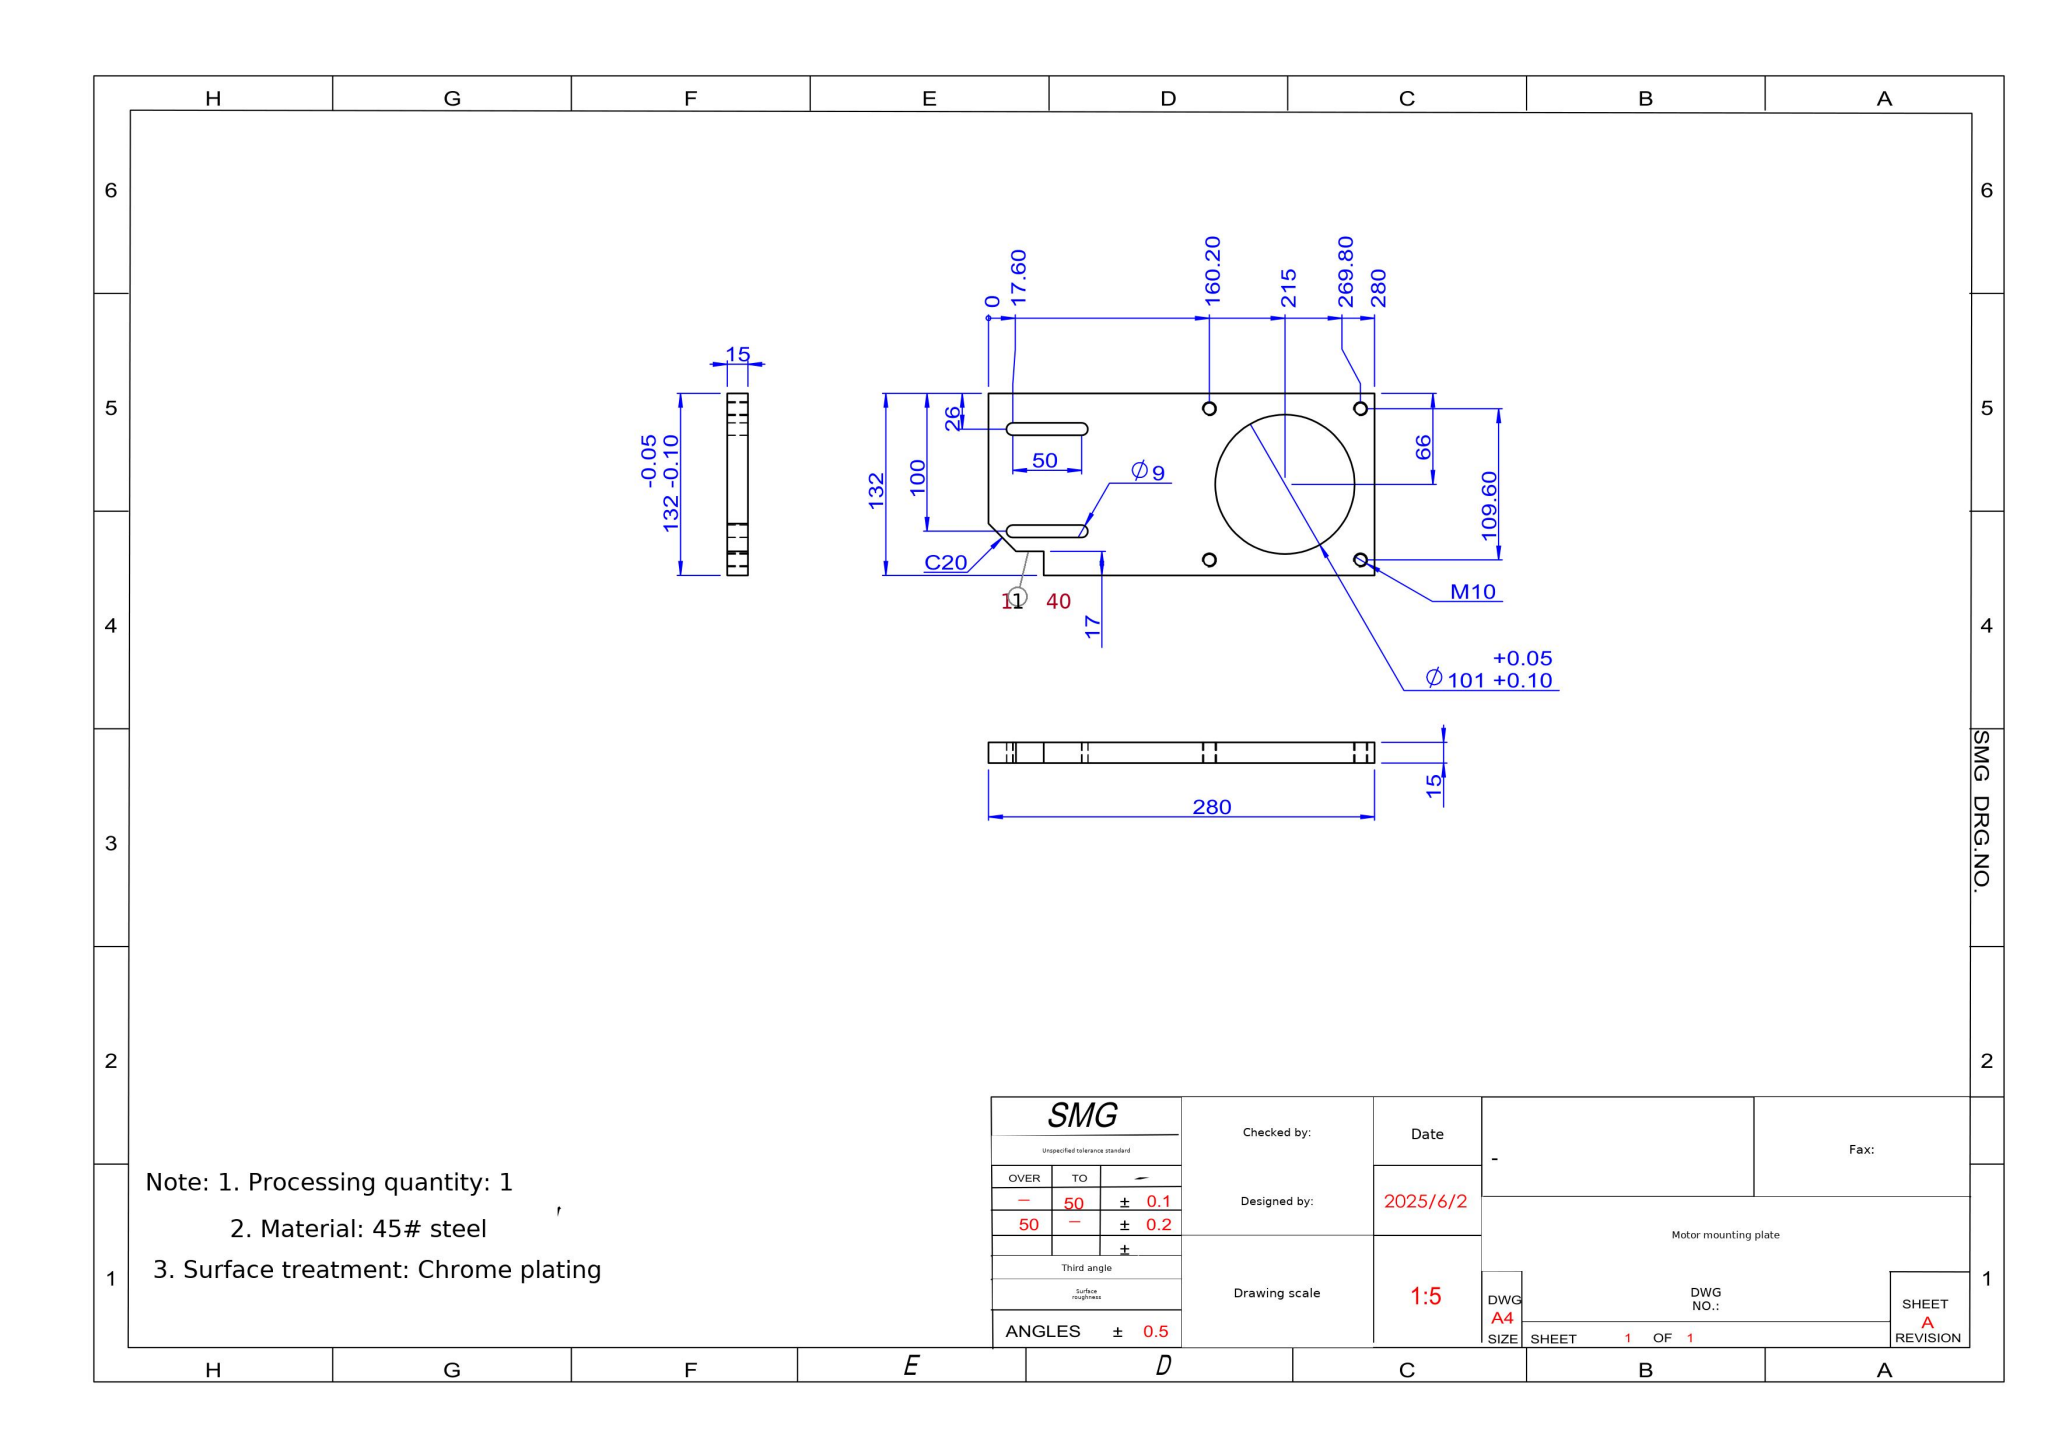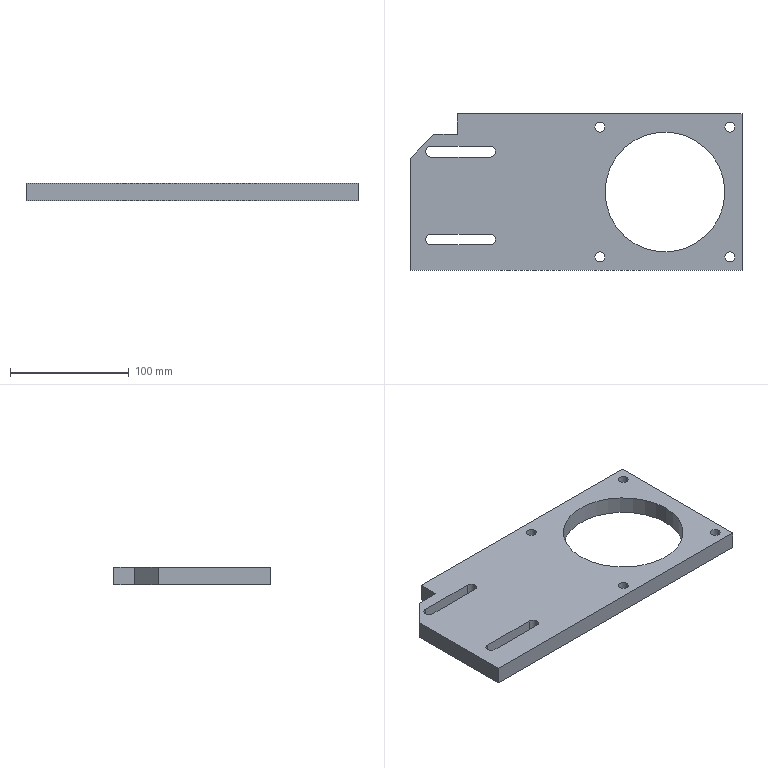Part | SolidWorks | mm | material 45# steel | 1 solid | 29 faces | box 280 x 132 x 15 mm | volume 401909 mm3 | cylinder 16 | plane 13 | commonest cylinder face diameters 8.5 x8 9 x6 101 x2
STEP:
#1=CARTESIAN_POINT('',(15.949,54.801,0.));
#2=VERTEX_POINT('',#1);
#3=CARTESIAN_POINT('',(24.449,54.801,0.));
#4=VERTEX_POINT('',#3);
#5=CARTESIAN_POINT('',(20.199,54.801,0.));
#6=DIRECTION('',(0.,0.,1.));
#7=DIRECTION('',(1.,0.,0.));
#8=AXIS2_PLACEMENT_3D('',#5,#6,#7);
#9=CIRCLE('',#8,4.25);
#10=EDGE_CURVE('',#2,#4,#9,.T.);
#11=ORIENTED_EDGE('',*,*,#10,.F.);
#12=CARTESIAN_POINT('',(15.949,54.801,15.));
#13=VERTEX_POINT('',#12);
#14=CARTESIAN_POINT('',(15.949,54.801,15.));
#15=DIRECTION('',(0.,0.,1.));
#16=VECTOR('',#15,1000.);
#17=LINE('',#14,#16);
#18=EDGE_CURVE('',#2,#13,#17,.T.);
#19=ORIENTED_EDGE('',*,*,#18,.T.);
#20=CARTESIAN_POINT('',(24.449,54.801,15.));
#21=VERTEX_POINT('',#20);
#22=CARTESIAN_POINT('',(20.199,54.801,15.));
#23=DIRECTION('',(0.,0.,-1.));
#24=DIRECTION('',(1.,0.,0.));
#25=AXIS2_PLACEMENT_3D('',#22,#23,#24);
#26=CIRCLE('',#25,4.25);
#27=EDGE_CURVE('',#21,#13,#26,.T.);
#28=ORIENTED_EDGE('',*,*,#27,.F.);
#29=CARTESIAN_POINT('',(24.449,54.801,15.));
#30=DIRECTION('',(0.,0.,1.));
#31=VECTOR('',#30,1000.);
#32=LINE('',#29,#31);
#33=EDGE_CURVE('',#4,#21,#32,.T.);
#34=ORIENTED_EDGE('',*,*,#33,.F.);
#35=EDGE_LOOP('',(#11,#19,#28,#34));
#36=FACE_OUTER_BOUND('',#35,.T.);
#37=CARTESIAN_POINT('',(20.199,54.801,15.));
#38=DIRECTION('',(0.,0.,1.));
#39=DIRECTION('',(1.,0.,0.));
#40=AXIS2_PLACEMENT_3D('',#37,#38,#39);
#41=CYLINDRICAL_SURFACE('',#40,4.25);
#42=ADVANCED_FACE('',(#36),#41,.F.);
#43=CARTESIAN_POINT('',(15.949,-54.801,0.));
#44=VERTEX_POINT('',#43);
#45=CARTESIAN_POINT('',(24.449,-54.801,0.));
#46=VERTEX_POINT('',#45);
#47=CARTESIAN_POINT('',(20.199,-54.801,0.));
#48=DIRECTION('',(0.,0.,1.));
#49=DIRECTION('',(1.,0.,0.));
#50=AXIS2_PLACEMENT_3D('',#47,#48,#49);
#51=CIRCLE('',#50,4.25);
#52=EDGE_CURVE('',#44,#46,#51,.T.);
#53=ORIENTED_EDGE('',*,*,#52,.F.);
#54=CARTESIAN_POINT('',(15.949,-54.801,15.));
#55=VERTEX_POINT('',#54);
#56=CARTESIAN_POINT('',(15.949,-54.801,15.));
#57=DIRECTION('',(0.,0.,1.));
#58=VECTOR('',#57,1000.);
#59=LINE('',#56,#58);
#60=EDGE_CURVE('',#44,#55,#59,.T.);
#61=ORIENTED_EDGE('',*,*,#60,.T.);
#62=CARTESIAN_POINT('',(24.449,-54.801,15.));
#63=VERTEX_POINT('',#62);
#64=CARTESIAN_POINT('',(20.199,-54.801,15.));
#65=DIRECTION('',(0.,0.,-1.));
#66=DIRECTION('',(1.,0.,0.));
#67=AXIS2_PLACEMENT_3D('',#64,#65,#66);
#68=CIRCLE('',#67,4.25);
#69=EDGE_CURVE('',#63,#55,#68,.T.);
#70=ORIENTED_EDGE('',*,*,#69,.F.);
#71=CARTESIAN_POINT('',(24.449,-54.801,15.));
#72=DIRECTION('',(0.,0.,1.));
#73=VECTOR('',#72,1000.);
#74=LINE('',#71,#73);
#75=EDGE_CURVE('',#46,#63,#74,.T.);
#76=ORIENTED_EDGE('',*,*,#75,.F.);
#77=EDGE_LOOP('',(#53,#61,#70,#76));
#78=FACE_OUTER_BOUND('',#77,.T.);
#79=CARTESIAN_POINT('',(20.199,-54.801,15.));
#80=DIRECTION('',(0.,0.,1.));
#81=DIRECTION('',(1.,0.,0.));
#82=AXIS2_PLACEMENT_3D('',#79,#80,#81);
#83=CYLINDRICAL_SURFACE('',#82,4.25);
#84=ADVANCED_FACE('',(#78),#83,.F.);
#85=CARTESIAN_POINT('',(125.551,-54.801,0.));
#86=VERTEX_POINT('',#85);
#87=CARTESIAN_POINT('',(134.051,-54.801,0.));
#88=VERTEX_POINT('',#87);
#89=CARTESIAN_POINT('',(129.801,-54.801,0.));
#90=DIRECTION('',(0.,0.,1.));
#91=DIRECTION('',(1.,0.,0.));
#92=AXIS2_PLACEMENT_3D('',#89,#90,#91);
#93=CIRCLE('',#92,4.25);
#94=EDGE_CURVE('',#86,#88,#93,.T.);
#95=ORIENTED_EDGE('',*,*,#94,.F.);
#96=CARTESIAN_POINT('',(125.551,-54.801,15.));
#97=VERTEX_POINT('',#96);
#98=CARTESIAN_POINT('',(125.551,-54.801,15.));
#99=DIRECTION('',(0.,0.,1.));
#100=VECTOR('',#99,1000.);
#101=LINE('',#98,#100);
#102=EDGE_CURVE('',#86,#97,#101,.T.);
#103=ORIENTED_EDGE('',*,*,#102,.T.);
#104=CARTESIAN_POINT('',(134.051,-54.801,15.));
#105=VERTEX_POINT('',#104);
#106=CARTESIAN_POINT('',(129.801,-54.801,15.));
#107=DIRECTION('',(0.,0.,-1.));
#108=DIRECTION('',(1.,0.,0.));
#109=AXIS2_PLACEMENT_3D('',#106,#107,#108);
#110=CIRCLE('',#109,4.25);
#111=EDGE_CURVE('',#105,#97,#110,.T.);
#112=ORIENTED_EDGE('',*,*,#111,.F.);
#113=CARTESIAN_POINT('',(134.051,-54.801,15.));
#114=DIRECTION('',(0.,0.,1.));
#115=VECTOR('',#114,1000.);
#116=LINE('',#113,#115);
#117=EDGE_CURVE('',#88,#105,#116,.T.);
#118=ORIENTED_EDGE('',*,*,#117,.F.);
#119=EDGE_LOOP('',(#95,#103,#112,#118));
#120=FACE_OUTER_BOUND('',#119,.T.);
#121=CARTESIAN_POINT('',(129.801,-54.801,15.));
#122=DIRECTION('',(0.,0.,1.));
#123=DIRECTION('',(1.,0.,0.));
#124=AXIS2_PLACEMENT_3D('',#121,#122,#123);
#125=CYLINDRICAL_SURFACE('',#124,4.25);
#126=ADVANCED_FACE('',(#120),#125,.F.);
#127=CARTESIAN_POINT('',(125.551,54.801,0.));
#128=VERTEX_POINT('',#127);
#129=CARTESIAN_POINT('',(134.051,54.801,0.));
#130=VERTEX_POINT('',#129);
#131=CARTESIAN_POINT('',(129.801,54.801,0.));
#132=DIRECTION('',(0.,0.,1.));
#133=DIRECTION('',(1.,0.,0.));
#134=AXIS2_PLACEMENT_3D('',#131,#132,#133);
#135=CIRCLE('',#134,4.25);
#136=EDGE_CURVE('',#128,#130,#135,.T.);
#137=ORIENTED_EDGE('',*,*,#136,.F.);
#138=CARTESIAN_POINT('',(125.551,54.801,15.));
#139=VERTEX_POINT('',#138);
#140=CARTESIAN_POINT('',(125.551,54.801,15.));
#141=DIRECTION('',(0.,0.,1.));
#142=VECTOR('',#141,1000.);
#143=LINE('',#140,#142);
#144=EDGE_CURVE('',#128,#139,#143,.T.);
#145=ORIENTED_EDGE('',*,*,#144,.T.);
#146=CARTESIAN_POINT('',(134.051,54.801,15.));
#147=VERTEX_POINT('',#146);
#148=CARTESIAN_POINT('',(129.801,54.801,15.));
#149=DIRECTION('',(0.,0.,-1.));
#150=DIRECTION('',(1.,0.,0.));
#151=AXIS2_PLACEMENT_3D('',#148,#149,#150);
#152=CIRCLE('',#151,4.25);
#153=EDGE_CURVE('',#147,#139,#152,.T.);
#154=ORIENTED_EDGE('',*,*,#153,.F.);
#155=CARTESIAN_POINT('',(134.051,54.801,15.));
#156=DIRECTION('',(0.,0.,1.));
#157=VECTOR('',#156,1000.);
#158=LINE('',#155,#157);
#159=EDGE_CURVE('',#130,#147,#158,.T.);
#160=ORIENTED_EDGE('',*,*,#159,.F.);
#161=EDGE_LOOP('',(#137,#145,#154,#160));
#162=FACE_OUTER_BOUND('',#161,.T.);
#163=CARTESIAN_POINT('',(129.801,54.801,15.));
#164=DIRECTION('',(0.,0.,1.));
#165=DIRECTION('',(1.,0.,0.));
#166=AXIS2_PLACEMENT_3D('',#163,#164,#165);
#167=CYLINDRICAL_SURFACE('',#166,4.25);
#168=ADVANCED_FACE('',(#162),#167,.F.);
#169=CARTESIAN_POINT('',(125.5,0.,15.));
#170=VERTEX_POINT('',#169);
#171=CARTESIAN_POINT('',(24.5,0.,15.));
#172=VERTEX_POINT('',#171);
#173=CARTESIAN_POINT('',(75.,0.,15.));
#174=DIRECTION('',(0.,0.,-1.));
#175=DIRECTION('',(-1.,0.,0.));
#176=AXIS2_PLACEMENT_3D('',#173,#174,#175);
#177=CIRCLE('',#176,50.5);
#178=EDGE_CURVE('',#170,#172,#177,.T.);
#179=ORIENTED_EDGE('',*,*,#178,.F.);
#180=CARTESIAN_POINT('',(125.5,0.,0.));
#181=VERTEX_POINT('',#180);
#182=CARTESIAN_POINT('',(125.5,0.,15.));
#183=DIRECTION('',(0.,0.,-1.));
#184=VECTOR('',#183,1000.);
#185=LINE('',#182,#184);
#186=EDGE_CURVE('',#170,#181,#185,.T.);
#187=ORIENTED_EDGE('',*,*,#186,.T.);
#188=CARTESIAN_POINT('',(24.5,0.,0.));
#189=VERTEX_POINT('',#188);
#190=CARTESIAN_POINT('',(75.,0.,0.));
#191=DIRECTION('',(0.,0.,1.));
#192=DIRECTION('',(-1.,0.,0.));
#193=AXIS2_PLACEMENT_3D('',#190,#191,#192);
#194=CIRCLE('',#193,50.5);
#195=EDGE_CURVE('',#189,#181,#194,.T.);
#196=ORIENTED_EDGE('',*,*,#195,.F.);
#197=CARTESIAN_POINT('',(24.5,0.,15.));
#198=DIRECTION('',(0.,0.,-1.));
#199=VECTOR('',#198,1000.);
#200=LINE('',#197,#199);
#201=EDGE_CURVE('',#172,#189,#200,.T.);
#202=ORIENTED_EDGE('',*,*,#201,.F.);
#203=EDGE_LOOP('',(#179,#187,#196,#202));
#204=FACE_OUTER_BOUND('',#203,.T.);
#205=CARTESIAN_POINT('',(75.,0.,15.));
#206=DIRECTION('',(0.,0.,-1.));
#207=DIRECTION('',(-1.,0.,0.));
#208=AXIS2_PLACEMENT_3D('',#205,#206,#207);
#209=CYLINDRICAL_SURFACE('',#208,50.5);
#210=ADVANCED_FACE('',(#204),#209,.F.);
#211=CARTESIAN_POINT('',(-126.902,34.,15.));
#212=VERTEX_POINT('',#211);
#213=CARTESIAN_POINT('',(-122.402,38.5,15.));
#214=VERTEX_POINT('',#213);
#215=CARTESIAN_POINT('',(-122.402,34.,15.));
#216=DIRECTION('',(0.,0.,-1.));
#217=DIRECTION('',(-1.,0.,0.));
#218=AXIS2_PLACEMENT_3D('',#215,#216,#217);
#219=CIRCLE('',#218,4.5);
#220=EDGE_CURVE('',#212,#214,#219,.T.);
#221=ORIENTED_EDGE('',*,*,#220,.F.);
#222=CARTESIAN_POINT('',(-126.902,34.,0.));
#223=VERTEX_POINT('',#222);
#224=CARTESIAN_POINT('',(-126.902,34.,15.));
#225=DIRECTION('',(0.,0.,-1.));
#226=VECTOR('',#225,1000.);
#227=LINE('',#224,#226);
#228=EDGE_CURVE('',#212,#223,#227,.T.);
#229=ORIENTED_EDGE('',*,*,#228,.T.);
#230=CARTESIAN_POINT('',(-122.402,38.5,0.));
#231=VERTEX_POINT('',#230);
#232=CARTESIAN_POINT('',(-122.402,34.,0.));
#233=DIRECTION('',(0.,0.,1.));
#234=DIRECTION('',(-1.,0.,0.));
#235=AXIS2_PLACEMENT_3D('',#232,#233,#234);
#236=CIRCLE('',#235,4.5);
#237=EDGE_CURVE('',#231,#223,#236,.T.);
#238=ORIENTED_EDGE('',*,*,#237,.F.);
#239=CARTESIAN_POINT('',(-122.402,38.5,15.));
#240=DIRECTION('',(0.,0.,1.));
#241=VECTOR('',#240,1000.);
#242=LINE('',#239,#241);
#243=EDGE_CURVE('',#231,#214,#242,.T.);
#244=ORIENTED_EDGE('',*,*,#243,.T.);
#245=EDGE_LOOP('',(#221,#229,#238,#244));
#246=FACE_OUTER_BOUND('',#245,.T.);
#247=CARTESIAN_POINT('',(-122.402,34.,15.));
#248=DIRECTION('',(0.,0.,-1.));
#249=DIRECTION('',(-1.,0.,0.));
#250=AXIS2_PLACEMENT_3D('',#247,#248,#249);
#251=CYLINDRICAL_SURFACE('',#250,4.5);
#252=ADVANCED_FACE('',(#246),#251,.F.);
#253=CARTESIAN_POINT('',(-126.902,-40.,15.));
#254=VERTEX_POINT('',#253);
#255=CARTESIAN_POINT('',(-122.402,-35.5,15.));
#256=VERTEX_POINT('',#255);
#257=CARTESIAN_POINT('',(-122.402,-40.,15.));
#258=DIRECTION('',(0.,0.,-1.));
#259=DIRECTION('',(-1.,0.,0.));
#260=AXIS2_PLACEMENT_3D('',#257,#258,#259);
#261=CIRCLE('',#260,4.5);
#262=EDGE_CURVE('',#254,#256,#261,.T.);
#263=ORIENTED_EDGE('',*,*,#262,.F.);
#264=CARTESIAN_POINT('',(-126.902,-40.,0.));
#265=VERTEX_POINT('',#264);
#266=CARTESIAN_POINT('',(-126.902,-40.,15.));
#267=DIRECTION('',(0.,0.,-1.));
#268=VECTOR('',#267,1000.);
#269=LINE('',#266,#268);
#270=EDGE_CURVE('',#254,#265,#269,.T.);
#271=ORIENTED_EDGE('',*,*,#270,.T.);
#272=CARTESIAN_POINT('',(-122.402,-35.5,0.));
#273=VERTEX_POINT('',#272);
#274=CARTESIAN_POINT('',(-122.402,-40.,0.));
#275=DIRECTION('',(0.,0.,1.));
#276=DIRECTION('',(-1.,0.,0.));
#277=AXIS2_PLACEMENT_3D('',#274,#275,#276);
#278=CIRCLE('',#277,4.5);
#279=EDGE_CURVE('',#273,#265,#278,.T.);
#280=ORIENTED_EDGE('',*,*,#279,.F.);
#281=CARTESIAN_POINT('',(-122.402,-35.5,15.));
#282=DIRECTION('',(0.,0.,1.));
#283=VECTOR('',#282,1000.);
#284=LINE('',#281,#283);
#285=EDGE_CURVE('',#273,#256,#284,.T.);
#286=ORIENTED_EDGE('',*,*,#285,.T.);
#287=EDGE_LOOP('',(#263,#271,#280,#286));
#288=FACE_OUTER_BOUND('',#287,.T.);
#289=CARTESIAN_POINT('',(-122.402,-40.,15.));
#290=DIRECTION('',(0.,0.,-1.));
#291=DIRECTION('',(-1.,0.,0.));
#292=AXIS2_PLACEMENT_3D('',#289,#290,#291);
#293=CYLINDRICAL_SURFACE('',#292,4.5);
#294=ADVANCED_FACE('',(#288),#293,.F.);
#295=ORIENTED_EDGE('',*,*,#27,.T.);
#296=CARTESIAN_POINT('',(20.199,54.801,15.));
#297=DIRECTION('',(0.,0.,-1.));
#298=DIRECTION('',(1.,0.,0.));
#299=AXIS2_PLACEMENT_3D('',#296,#297,#298);
#300=CIRCLE('',#299,4.25);
#301=EDGE_CURVE('',#13,#21,#300,.T.);
#302=ORIENTED_EDGE('',*,*,#301,.T.);
#303=EDGE_LOOP('',(#295,#302));
#304=FACE_BOUND('',#303,.T.);
#305=ORIENTED_EDGE('',*,*,#69,.T.);
#306=CARTESIAN_POINT('',(20.199,-54.801,15.));
#307=DIRECTION('',(0.,0.,-1.));
#308=DIRECTION('',(1.,0.,0.));
#309=AXIS2_PLACEMENT_3D('',#306,#307,#308);
#310=CIRCLE('',#309,4.25);
#311=EDGE_CURVE('',#55,#63,#310,.T.);
#312=ORIENTED_EDGE('',*,*,#311,.T.);
#313=EDGE_LOOP('',(#305,#312));
#314=FACE_BOUND('',#313,.T.);
#315=ORIENTED_EDGE('',*,*,#111,.T.);
#316=CARTESIAN_POINT('',(129.801,-54.801,15.));
#317=DIRECTION('',(0.,0.,-1.));
#318=DIRECTION('',(1.,0.,0.));
#319=AXIS2_PLACEMENT_3D('',#316,#317,#318);
#320=CIRCLE('',#319,4.25);
#321=EDGE_CURVE('',#97,#105,#320,.T.);
#322=ORIENTED_EDGE('',*,*,#321,.T.);
#323=EDGE_LOOP('',(#315,#322));
#324=FACE_BOUND('',#323,.T.);
#325=ORIENTED_EDGE('',*,*,#153,.T.);
#326=CARTESIAN_POINT('',(129.801,54.801,15.));
#327=DIRECTION('',(0.,0.,-1.));
#328=DIRECTION('',(1.,0.,0.));
#329=AXIS2_PLACEMENT_3D('',#326,#327,#328);
#330=CIRCLE('',#329,4.25);
#331=EDGE_CURVE('',#139,#147,#330,.T.);
#332=ORIENTED_EDGE('',*,*,#331,.T.);
#333=EDGE_LOOP('',(#325,#332));
#334=FACE_BOUND('',#333,.T.);
#335=CARTESIAN_POINT('',(75.,0.,15.));
#336=DIRECTION('',(0.,0.,-1.));
#337=DIRECTION('',(-1.,0.,0.));
#338=AXIS2_PLACEMENT_3D('',#335,#336,#337);
#339=CIRCLE('',#338,50.5);
#340=EDGE_CURVE('',#172,#170,#339,.T.);
#341=ORIENTED_EDGE('',*,*,#340,.T.);
#342=ORIENTED_EDGE('',*,*,#178,.T.);
#343=EDGE_LOOP('',(#341,#342));
#344=FACE_BOUND('',#343,.T.);
#345=CARTESIAN_POINT('',(-122.402,29.5,15.));
#346=VERTEX_POINT('',#345);
#347=CARTESIAN_POINT('',(-122.402,34.,15.));
#348=DIRECTION('',(0.,0.,-1.));
#349=DIRECTION('',(-1.,0.,0.));
#350=AXIS2_PLACEMENT_3D('',#347,#348,#349);
#351=CIRCLE('',#350,4.5);
#352=EDGE_CURVE('',#346,#212,#351,.T.);
#353=ORIENTED_EDGE('',*,*,#352,.T.);
#354=ORIENTED_EDGE('',*,*,#220,.T.);
#355=CARTESIAN_POINT('',(-72.402,38.5,15.));
#356=VERTEX_POINT('',#355);
#357=CARTESIAN_POINT('',(0.,38.5,15.));
#358=DIRECTION('',(1.,0.,0.));
#359=VECTOR('',#358,1000.);
#360=LINE('',#357,#359);
#361=EDGE_CURVE('',#214,#356,#360,.T.);
#362=ORIENTED_EDGE('',*,*,#361,.T.);
#363=CARTESIAN_POINT('',(-72.402,29.5,15.));
#364=VERTEX_POINT('',#363);
#365=CARTESIAN_POINT('',(-72.402,34.,15.));
#366=DIRECTION('',(0.,0.,-1.));
#367=DIRECTION('',(-1.,0.,0.));
#368=AXIS2_PLACEMENT_3D('',#365,#366,#367);
#369=CIRCLE('',#368,4.5);
#370=EDGE_CURVE('',#356,#364,#369,.T.);
#371=ORIENTED_EDGE('',*,*,#370,.T.);
#372=CARTESIAN_POINT('',(0.,29.5,15.));
#373=DIRECTION('',(-1.,0.,0.));
#374=VECTOR('',#373,1000.);
#375=LINE('',#372,#374);
#376=EDGE_CURVE('',#364,#346,#375,.T.);
#377=ORIENTED_EDGE('',*,*,#376,.T.);
#378=EDGE_LOOP('',(#353,#354,#362,#371,#377));
#379=FACE_BOUND('',#378,.T.);
#380=CARTESIAN_POINT('',(-72.402,-35.5,15.));
#381=VERTEX_POINT('',#380);
#382=CARTESIAN_POINT('',(-72.402,-44.5,15.));
#383=VERTEX_POINT('',#382);
#384=CARTESIAN_POINT('',(-72.402,-40.,15.));
#385=DIRECTION('',(0.,0.,-1.));
#386=DIRECTION('',(-1.,0.,0.));
#387=AXIS2_PLACEMENT_3D('',#384,#385,#386);
#388=CIRCLE('',#387,4.5);
#389=EDGE_CURVE('',#381,#383,#388,.T.);
#390=ORIENTED_EDGE('',*,*,#389,.T.);
#391=CARTESIAN_POINT('',(-122.402,-44.5,15.));
#392=VERTEX_POINT('',#391);
#393=CARTESIAN_POINT('',(0.,-44.5,15.));
#394=DIRECTION('',(-1.,0.,0.));
#395=VECTOR('',#394,1000.);
#396=LINE('',#393,#395);
#397=EDGE_CURVE('',#383,#392,#396,.T.);
#398=ORIENTED_EDGE('',*,*,#397,.T.);
#399=CARTESIAN_POINT('',(-122.402,-40.,15.));
#400=DIRECTION('',(0.,0.,-1.));
#401=DIRECTION('',(-1.,0.,0.));
#402=AXIS2_PLACEMENT_3D('',#399,#400,#401);
#403=CIRCLE('',#402,4.5);
#404=EDGE_CURVE('',#392,#254,#403,.T.);
#405=ORIENTED_EDGE('',*,*,#404,.T.);
#406=ORIENTED_EDGE('',*,*,#262,.T.);
#407=CARTESIAN_POINT('',(0.,-35.5,15.));
#408=DIRECTION('',(1.,0.,0.));
#409=VECTOR('',#408,1000.);
#410=LINE('',#407,#409);
#411=EDGE_CURVE('',#256,#381,#410,.T.);
#412=ORIENTED_EDGE('',*,*,#411,.T.);
#413=EDGE_LOOP('',(#390,#398,#405,#406,#412));
#414=FACE_BOUND('',#413,.T.);
#415=CARTESIAN_POINT('',(140.,66.,15.));
#416=VERTEX_POINT('',#415);
#417=CARTESIAN_POINT('',(-100.,66.,15.));
#418=VERTEX_POINT('',#417);
#419=CARTESIAN_POINT('',(0.,66.,15.));
#420=DIRECTION('',(-1.,0.,0.));
#421=VECTOR('',#420,1000.);
#422=LINE('',#419,#421);
#423=EDGE_CURVE('',#416,#418,#422,.T.);
#424=ORIENTED_EDGE('',*,*,#423,.T.);
#425=CARTESIAN_POINT('',(-100.,48.5,15.));
#426=VERTEX_POINT('',#425);
#427=CARTESIAN_POINT('',(-100.,0.,15.));
#428=DIRECTION('',(0.,-1.,0.));
#429=VECTOR('',#428,1000.);
#430=LINE('',#427,#429);
#431=EDGE_CURVE('',#418,#426,#430,.T.);
#432=ORIENTED_EDGE('',*,*,#431,.T.);
#433=CARTESIAN_POINT('',(-120.,48.5,15.));
#434=VERTEX_POINT('',#433);
#435=CARTESIAN_POINT('',(0.,48.5,15.));
#436=DIRECTION('',(-1.,0.,0.));
#437=VECTOR('',#436,1000.);
#438=LINE('',#435,#437);
#439=EDGE_CURVE('',#426,#434,#438,.T.);
#440=ORIENTED_EDGE('',*,*,#439,.T.);
#441=CARTESIAN_POINT('',(-140.,28.5,15.));
#442=VERTEX_POINT('',#441);
#443=CARTESIAN_POINT('',(-120.,48.5,15.));
#444=DIRECTION('',(-0.7071,-0.7071,0.));
#445=VECTOR('',#444,1000.);
#446=LINE('',#443,#445);
#447=EDGE_CURVE('',#434,#442,#446,.T.);
#448=ORIENTED_EDGE('',*,*,#447,.T.);
#449=CARTESIAN_POINT('',(-140.,-66.,15.));
#450=VERTEX_POINT('',#449);
#451=CARTESIAN_POINT('',(-140.,0.,15.));
#452=DIRECTION('',(0.,-1.,0.));
#453=VECTOR('',#452,1000.);
#454=LINE('',#451,#453);
#455=EDGE_CURVE('',#442,#450,#454,.T.);
#456=ORIENTED_EDGE('',*,*,#455,.T.);
#457=CARTESIAN_POINT('',(140.,-66.,15.));
#458=VERTEX_POINT('',#457);
#459=CARTESIAN_POINT('',(0.,-66.,15.));
#460=DIRECTION('',(1.,0.,0.));
#461=VECTOR('',#460,1000.);
#462=LINE('',#459,#461);
#463=EDGE_CURVE('',#450,#458,#462,.T.);
#464=ORIENTED_EDGE('',*,*,#463,.T.);
#465=CARTESIAN_POINT('',(140.,0.,15.));
#466=DIRECTION('',(0.,1.,0.));
#467=VECTOR('',#466,1000.);
#468=LINE('',#465,#467);
#469=EDGE_CURVE('',#458,#416,#468,.T.);
#470=ORIENTED_EDGE('',*,*,#469,.T.);
#471=EDGE_LOOP('',(#424,#432,#440,#448,#456,#464,#470));
#472=FACE_OUTER_BOUND('',#471,.T.);
#473=CARTESIAN_POINT('',(0.,0.,15.));
#474=DIRECTION('',(0.,0.,1.));
#475=DIRECTION('',(1.,0.,0.));
#476=AXIS2_PLACEMENT_3D('',#473,#474,#475);
#477=PLANE('',#476);
#478=ADVANCED_FACE('',(#304,#314,#324,#334,#344,#379,#414,#472),#477,.T.);
#479=ORIENTED_EDGE('',*,*,#18,.F.);
#480=CARTESIAN_POINT('',(20.199,54.801,0.));
#481=DIRECTION('',(0.,0.,1.));
#482=DIRECTION('',(1.,0.,0.));
#483=AXIS2_PLACEMENT_3D('',#480,#481,#482);
#484=CIRCLE('',#483,4.25);
#485=EDGE_CURVE('',#4,#2,#484,.T.);
#486=ORIENTED_EDGE('',*,*,#485,.F.);
#487=ORIENTED_EDGE('',*,*,#33,.T.);
#488=ORIENTED_EDGE('',*,*,#301,.F.);
#489=EDGE_LOOP('',(#479,#486,#487,#488));
#490=FACE_OUTER_BOUND('',#489,.T.);
#491=CARTESIAN_POINT('',(20.199,54.801,15.));
#492=DIRECTION('',(0.,0.,1.));
#493=DIRECTION('',(1.,0.,0.));
#494=AXIS2_PLACEMENT_3D('',#491,#492,#493);
#495=CYLINDRICAL_SURFACE('',#494,4.25);
#496=ADVANCED_FACE('',(#490),#495,.F.);
#497=ORIENTED_EDGE('',*,*,#60,.F.);
#498=CARTESIAN_POINT('',(20.199,-54.801,0.));
#499=DIRECTION('',(0.,0.,1.));
#500=DIRECTION('',(1.,0.,0.));
#501=AXIS2_PLACEMENT_3D('',#498,#499,#500);
#502=CIRCLE('',#501,4.25);
#503=EDGE_CURVE('',#46,#44,#502,.T.);
#504=ORIENTED_EDGE('',*,*,#503,.F.);
#505=ORIENTED_EDGE('',*,*,#75,.T.);
#506=ORIENTED_EDGE('',*,*,#311,.F.);
#507=EDGE_LOOP('',(#497,#504,#505,#506));
#508=FACE_OUTER_BOUND('',#507,.T.);
#509=CARTESIAN_POINT('',(20.199,-54.801,15.));
#510=DIRECTION('',(0.,0.,1.));
#511=DIRECTION('',(1.,0.,0.));
#512=AXIS2_PLACEMENT_3D('',#509,#510,#511);
#513=CYLINDRICAL_SURFACE('',#512,4.25);
#514=ADVANCED_FACE('',(#508),#513,.F.);
#515=ORIENTED_EDGE('',*,*,#102,.F.);
#516=CARTESIAN_POINT('',(129.801,-54.801,0.));
#517=DIRECTION('',(0.,0.,1.));
#518=DIRECTION('',(1.,0.,0.));
#519=AXIS2_PLACEMENT_3D('',#516,#517,#518);
#520=CIRCLE('',#519,4.25);
#521=EDGE_CURVE('',#88,#86,#520,.T.);
#522=ORIENTED_EDGE('',*,*,#521,.F.);
#523=ORIENTED_EDGE('',*,*,#117,.T.);
#524=ORIENTED_EDGE('',*,*,#321,.F.);
#525=EDGE_LOOP('',(#515,#522,#523,#524));
#526=FACE_OUTER_BOUND('',#525,.T.);
#527=CARTESIAN_POINT('',(129.801,-54.801,15.));
#528=DIRECTION('',(0.,0.,1.));
#529=DIRECTION('',(1.,0.,0.));
#530=AXIS2_PLACEMENT_3D('',#527,#528,#529);
#531=CYLINDRICAL_SURFACE('',#530,4.25);
#532=ADVANCED_FACE('',(#526),#531,.F.);
#533=ORIENTED_EDGE('',*,*,#144,.F.);
#534=CARTESIAN_POINT('',(129.801,54.801,0.));
#535=DIRECTION('',(0.,0.,1.));
#536=DIRECTION('',(1.,0.,0.));
#537=AXIS2_PLACEMENT_3D('',#534,#535,#536);
#538=CIRCLE('',#537,4.25);
#539=EDGE_CURVE('',#130,#128,#538,.T.);
#540=ORIENTED_EDGE('',*,*,#539,.F.);
#541=ORIENTED_EDGE('',*,*,#159,.T.);
#542=ORIENTED_EDGE('',*,*,#331,.F.);
#543=EDGE_LOOP('',(#533,#540,#541,#542));
#544=FACE_OUTER_BOUND('',#543,.T.);
#545=CARTESIAN_POINT('',(129.801,54.801,15.));
#546=DIRECTION('',(0.,0.,1.));
#547=DIRECTION('',(1.,0.,0.));
#548=AXIS2_PLACEMENT_3D('',#545,#546,#547);
#549=CYLINDRICAL_SURFACE('',#548,4.25);
#550=ADVANCED_FACE('',(#544),#549,.F.);
#551=ORIENTED_EDGE('',*,*,#186,.F.);
#552=ORIENTED_EDGE('',*,*,#340,.F.);
#553=ORIENTED_EDGE('',*,*,#201,.T.);
#554=CARTESIAN_POINT('',(75.,0.,0.));
#555=DIRECTION('',(0.,0.,1.));
#556=DIRECTION('',(-1.,0.,0.));
#557=AXIS2_PLACEMENT_3D('',#554,#555,#556);
#558=CIRCLE('',#557,50.5);
#559=EDGE_CURVE('',#181,#189,#558,.T.);
#560=ORIENTED_EDGE('',*,*,#559,.F.);
#561=EDGE_LOOP('',(#551,#552,#553,#560));
#562=FACE_OUTER_BOUND('',#561,.T.);
#563=CARTESIAN_POINT('',(75.,0.,15.));
#564=DIRECTION('',(0.,0.,-1.));
#565=DIRECTION('',(-1.,0.,0.));
#566=AXIS2_PLACEMENT_3D('',#563,#564,#565);
#567=CYLINDRICAL_SURFACE('',#566,50.5);
#568=ADVANCED_FACE('',(#562),#567,.F.);
#569=CARTESIAN_POINT('',(-72.402,38.5,0.));
#570=VERTEX_POINT('',#569);
#571=CARTESIAN_POINT('',(-72.402,38.5,15.));
#572=DIRECTION('',(0.,0.,-1.));
#573=VECTOR('',#572,1000.);
#574=LINE('',#571,#573);
#575=EDGE_CURVE('',#356,#570,#574,.T.);
#576=ORIENTED_EDGE('',*,*,#575,.F.);
#577=ORIENTED_EDGE('',*,*,#361,.F.);
#578=ORIENTED_EDGE('',*,*,#243,.F.);
#579=CARTESIAN_POINT('',(-72.402,38.5,0.));
#580=DIRECTION('',(-1.,0.,0.));
#581=VECTOR('',#580,1000.);
#582=LINE('',#579,#581);
#583=EDGE_CURVE('',#570,#231,#582,.T.);
#584=ORIENTED_EDGE('',*,*,#583,.F.);
#585=EDGE_LOOP('',(#576,#577,#578,#584));
#586=FACE_OUTER_BOUND('',#585,.T.);
#587=CARTESIAN_POINT('',(-72.402,38.5,15.));
#588=DIRECTION('',(0.,1.,0.));
#589=DIRECTION('',(-1.,0.,0.));
#590=AXIS2_PLACEMENT_3D('',#587,#588,#589);
#591=PLANE('',#590);
#592=ADVANCED_FACE('',(#586),#591,.F.);
#593=ORIENTED_EDGE('',*,*,#228,.F.);
#594=ORIENTED_EDGE('',*,*,#352,.F.);
#595=CARTESIAN_POINT('',(-122.402,29.5,0.));
#596=VERTEX_POINT('',#595);
#597=CARTESIAN_POINT('',(-122.402,29.5,15.));
#598=DIRECTION('',(0.,0.,1.));
#599=VECTOR('',#598,1000.);
#600=LINE('',#597,#599);
#601=EDGE_CURVE('',#596,#346,#600,.T.);
#602=ORIENTED_EDGE('',*,*,#601,.F.);
#603=CARTESIAN_POINT('',(-122.402,34.,0.));
#604=DIRECTION('',(0.,0.,1.));
#605=DIRECTION('',(-1.,0.,0.));
#606=AXIS2_PLACEMENT_3D('',#603,#604,#605);
#607=CIRCLE('',#606,4.5);
#608=EDGE_CURVE('',#223,#596,#607,.T.);
#609=ORIENTED_EDGE('',*,*,#608,.F.);
#610=EDGE_LOOP('',(#593,#594,#602,#609));
#611=FACE_OUTER_BOUND('',#610,.T.);
#612=CARTESIAN_POINT('',(-122.402,34.,15.));
#613=DIRECTION('',(0.,0.,-1.));
#614=DIRECTION('',(-1.,0.,0.));
#615=AXIS2_PLACEMENT_3D('',#612,#613,#614);
#616=CYLINDRICAL_SURFACE('',#615,4.5);
#617=ADVANCED_FACE('',(#611),#616,.F.);
#618=ORIENTED_EDGE('',*,*,#601,.T.);
#619=ORIENTED_EDGE('',*,*,#376,.F.);
#620=CARTESIAN_POINT('',(-72.402,29.5,0.));
#621=VERTEX_POINT('',#620);
#622=CARTESIAN_POINT('',(-72.402,29.5,15.));
#623=DIRECTION('',(0.,0.,1.));
#624=VECTOR('',#623,1000.);
#625=LINE('',#622,#624);
#626=EDGE_CURVE('',#621,#364,#625,.T.);
#627=ORIENTED_EDGE('',*,*,#626,.F.);
#628=CARTESIAN_POINT('',(-72.402,29.5,0.));
#629=DIRECTION('',(1.,-0.,0.));
#630=VECTOR('',#629,1000.);
#631=LINE('',#628,#630);
#632=EDGE_CURVE('',#596,#621,#631,.T.);
#633=ORIENTED_EDGE('',*,*,#632,.F.);
#634=EDGE_LOOP('',(#618,#619,#627,#633));
#635=FACE_OUTER_BOUND('',#634,.T.);
#636=CARTESIAN_POINT('',(-72.402,29.5,15.));
#637=DIRECTION('',(-0.,-1.,0.));
#638=DIRECTION('',(1.,-0.,0.));
#639=AXIS2_PLACEMENT_3D('',#636,#637,#638);
#640=PLANE('',#639);
#641=ADVANCED_FACE('',(#635),#640,.F.);
#642=ORIENTED_EDGE('',*,*,#626,.T.);
#643=ORIENTED_EDGE('',*,*,#370,.F.);
#644=ORIENTED_EDGE('',*,*,#575,.T.);
#645=CARTESIAN_POINT('',(-72.402,34.,0.));
#646=DIRECTION('',(0.,0.,1.));
#647=DIRECTION('',(-1.,0.,0.));
#648=AXIS2_PLACEMENT_3D('',#645,#646,#647);
#649=CIRCLE('',#648,4.5);
#650=EDGE_CURVE('',#621,#570,#649,.T.);
#651=ORIENTED_EDGE('',*,*,#650,.F.);
#652=EDGE_LOOP('',(#642,#643,#644,#651));
#653=FACE_OUTER_BOUND('',#652,.T.);
#654=CARTESIAN_POINT('',(-72.402,34.,15.));
#655=DIRECTION('',(0.,0.,-1.));
#656=DIRECTION('',(-1.,0.,0.));
#657=AXIS2_PLACEMENT_3D('',#654,#655,#656);
#658=CYLINDRICAL_SURFACE('',#657,4.5);
#659=ADVANCED_FACE('',(#653),#658,.F.);
#660=CARTESIAN_POINT('',(-122.402,-44.5,0.));
#661=VERTEX_POINT('',#660);
#662=CARTESIAN_POINT('',(-122.402,-44.5,15.));
#663=DIRECTION('',(0.,0.,-1.));
#664=VECTOR('',#663,1000.);
#665=LINE('',#662,#664);
#666=EDGE_CURVE('',#392,#661,#665,.T.);
#667=ORIENTED_EDGE('',*,*,#666,.F.);
#668=ORIENTED_EDGE('',*,*,#397,.F.);
#669=CARTESIAN_POINT('',(-72.402,-44.5,0.));
#670=VERTEX_POINT('',#669);
#671=CARTESIAN_POINT('',(-72.402,-44.5,15.));
#672=DIRECTION('',(0.,0.,1.));
#673=VECTOR('',#672,1000.);
#674=LINE('',#671,#673);
#675=EDGE_CURVE('',#670,#383,#674,.T.);
#676=ORIENTED_EDGE('',*,*,#675,.F.);
#677=CARTESIAN_POINT('',(-122.402,-44.5,0.));
#678=DIRECTION('',(1.,0.,0.));
#679=VECTOR('',#678,1000.);
#680=LINE('',#677,#679);
#681=EDGE_CURVE('',#661,#670,#680,.T.);
#682=ORIENTED_EDGE('',*,*,#681,.F.);
#683=EDGE_LOOP('',(#667,#668,#676,#682));
#684=FACE_OUTER_BOUND('',#683,.T.);
#685=CARTESIAN_POINT('',(-122.402,-44.5,15.));
#686=DIRECTION('',(0.,-1.,0.));
#687=DIRECTION('',(0.,0.,-1.));
#688=AXIS2_PLACEMENT_3D('',#685,#686,#687);
#689=PLANE('',#688);
#690=ADVANCED_FACE('',(#684),#689,.F.);
#691=ORIENTED_EDGE('',*,*,#675,.T.);
#692=ORIENTED_EDGE('',*,*,#389,.F.);
#693=CARTESIAN_POINT('',(-72.402,-35.5,0.));
#694=VERTEX_POINT('',#693);
#695=CARTESIAN_POINT('',(-72.402,-35.5,15.));
#696=DIRECTION('',(0.,0.,1.));
#697=VECTOR('',#696,1000.);
#698=LINE('',#695,#697);
#699=EDGE_CURVE('',#694,#381,#698,.T.);
#700=ORIENTED_EDGE('',*,*,#699,.F.);
#701=CARTESIAN_POINT('',(-72.402,-40.,0.));
#702=DIRECTION('',(0.,0.,1.));
#703=DIRECTION('',(-1.,0.,0.));
#704=AXIS2_PLACEMENT_3D('',#701,#702,#703);
#705=CIRCLE('',#704,4.5);
#706=EDGE_CURVE('',#670,#694,#705,.T.);
#707=ORIENTED_EDGE('',*,*,#706,.F.);
#708=EDGE_LOOP('',(#691,#692,#700,#707));
#709=FACE_OUTER_BOUND('',#708,.T.);
#710=CARTESIAN_POINT('',(-72.402,-40.,15.));
#711=DIRECTION('',(0.,0.,-1.));
#712=DIRECTION('',(-1.,0.,0.));
#713=AXIS2_PLACEMENT_3D('',#710,#711,#712);
#714=CYLINDRICAL_SURFACE('',#713,4.5);
#715=ADVANCED_FACE('',(#709),#714,.F.);
#716=ORIENTED_EDGE('',*,*,#699,.T.);
#717=ORIENTED_EDGE('',*,*,#411,.F.);
#718=ORIENTED_EDGE('',*,*,#285,.F.);
#719=CARTESIAN_POINT('',(-122.402,-35.5,0.));
#720=DIRECTION('',(-1.,0.,0.));
#721=VECTOR('',#720,1000.);
#722=LINE('',#719,#721);
#723=EDGE_CURVE('',#694,#273,#722,.T.);
#724=ORIENTED_EDGE('',*,*,#723,.F.);
#725=EDGE_LOOP('',(#716,#717,#718,#724));
#726=FACE_OUTER_BOUND('',#725,.T.);
#727=CARTESIAN_POINT('',(-122.402,-35.5,15.));
#728=DIRECTION('',(0.,1.,0.));
#729=DIRECTION('',(-1.,0.,0.));
#730=AXIS2_PLACEMENT_3D('',#727,#728,#729);
#731=PLANE('',#730);
#732=ADVANCED_FACE('',(#726),#731,.F.);
#733=ORIENTED_EDGE('',*,*,#270,.F.);
#734=ORIENTED_EDGE('',*,*,#404,.F.);
#735=ORIENTED_EDGE('',*,*,#666,.T.);
#736=CARTESIAN_POINT('',(-122.402,-40.,0.));
#737=DIRECTION('',(0.,0.,1.));
#738=DIRECTION('',(-1.,0.,0.));
#739=AXIS2_PLACEMENT_3D('',#736,#737,#738);
#740=CIRCLE('',#739,4.5);
#741=EDGE_CURVE('',#265,#661,#740,.T.);
#742=ORIENTED_EDGE('',*,*,#741,.F.);
#743=EDGE_LOOP('',(#733,#734,#735,#742));
#744=FACE_OUTER_BOUND('',#743,.T.);
#745=CARTESIAN_POINT('',(-122.402,-40.,15.));
#746=DIRECTION('',(0.,0.,-1.));
#747=DIRECTION('',(-1.,0.,0.));
#748=AXIS2_PLACEMENT_3D('',#745,#746,#747);
#749=CYLINDRICAL_SURFACE('',#748,4.5);
#750=ADVANCED_FACE('',(#744),#749,.F.);
#751=CARTESIAN_POINT('',(-100.,66.,0.));
#752=VERTEX_POINT('',#751);
#753=CARTESIAN_POINT('',(-100.,66.,0.));
#754=DIRECTION('',(0.,0.,1.));
#755=VECTOR('',#754,1000.);
#756=LINE('',#753,#755);
#757=EDGE_CURVE('',#752,#418,#756,.T.);
#758=ORIENTED_EDGE('',*,*,#757,.F.);
#759=CARTESIAN_POINT('',(-100.,48.5,0.));
#760=VERTEX_POINT('',#759);
#761=CARTESIAN_POINT('',(-100.,66.,0.));
#762=DIRECTION('',(-0.,1.,0.));
#763=VECTOR('',#762,1000.);
#764=LINE('',#761,#763);
#765=EDGE_CURVE('',#760,#752,#764,.T.);
#766=ORIENTED_EDGE('',*,*,#765,.F.);
#767=CARTESIAN_POINT('',(-100.,48.5,0.));
#768=DIRECTION('',(0.,0.,-1.));
#769=VECTOR('',#768,1000.);
#770=LINE('',#767,#769);
#771=EDGE_CURVE('',#426,#760,#770,.T.);
#772=ORIENTED_EDGE('',*,*,#771,.F.);
#773=ORIENTED_EDGE('',*,*,#431,.F.);
#774=EDGE_LOOP('',(#758,#766,#772,#773));
#775=FACE_OUTER_BOUND('',#774,.T.);
#776=CARTESIAN_POINT('',(-100.,66.,0.));
#777=DIRECTION('',(1.,0.,0.));
#778=DIRECTION('',(-0.,1.,0.));
#779=AXIS2_PLACEMENT_3D('',#776,#777,#778);
#780=PLANE('',#779);
#781=ADVANCED_FACE('',(#775),#780,.F.);
#782=ORIENTED_EDGE('',*,*,#757,.T.);
#783=ORIENTED_EDGE('',*,*,#423,.F.);
#784=CARTESIAN_POINT('',(140.,66.,0.));
#785=VERTEX_POINT('',#784);
#786=CARTESIAN_POINT('',(140.,66.,15.));
#787=DIRECTION('',(0.,0.,1.));
#788=VECTOR('',#787,1000.);
#789=LINE('',#786,#788);
#790=EDGE_CURVE('',#785,#416,#789,.T.);
#791=ORIENTED_EDGE('',*,*,#790,.F.);
#792=CARTESIAN_POINT('',(140.,66.,0.));
#793=DIRECTION('',(1.,0.,0.));
#794=VECTOR('',#793,1000.);
#795=LINE('',#792,#794);
#796=EDGE_CURVE('',#752,#785,#795,.T.);
#797=ORIENTED_EDGE('',*,*,#796,.F.);
#798=EDGE_LOOP('',(#782,#783,#791,#797));
#799=FACE_OUTER_BOUND('',#798,.T.);
#800=CARTESIAN_POINT('',(140.,66.,15.));
#801=DIRECTION('',(0.,-1.,0.));
#802=DIRECTION('',(1.,0.,0.));
#803=AXIS2_PLACEMENT_3D('',#800,#801,#802);
#804=PLANE('',#803);
#805=ADVANCED_FACE('',(#799),#804,.F.);
#806=ORIENTED_EDGE('',*,*,#790,.T.);
#807=ORIENTED_EDGE('',*,*,#469,.F.);
#808=CARTESIAN_POINT('',(140.,-66.,0.));
#809=VERTEX_POINT('',#808);
#810=CARTESIAN_POINT('',(140.,-66.,15.));
#811=DIRECTION('',(0.,0.,1.));
#812=VECTOR('',#811,1000.);
#813=LINE('',#810,#812);
#814=EDGE_CURVE('',#809,#458,#813,.T.);
#815=ORIENTED_EDGE('',*,*,#814,.F.);
#816=CARTESIAN_POINT('',(140.,-66.,0.));
#817=DIRECTION('',(0.,-1.,0.));
#818=VECTOR('',#817,1000.);
#819=LINE('',#816,#818);
#820=EDGE_CURVE('',#785,#809,#819,.T.);
#821=ORIENTED_EDGE('',*,*,#820,.F.);
#822=EDGE_LOOP('',(#806,#807,#815,#821));
#823=FACE_OUTER_BOUND('',#822,.T.);
#824=CARTESIAN_POINT('',(140.,-66.,15.));
#825=DIRECTION('',(-1.,0.,0.));
#826=DIRECTION('',(0.,0.,1.));
#827=AXIS2_PLACEMENT_3D('',#824,#825,#826);
#828=PLANE('',#827);
#829=ADVANCED_FACE('',(#823),#828,.F.);
#830=ORIENTED_EDGE('',*,*,#814,.T.);
#831=ORIENTED_EDGE('',*,*,#463,.F.);
#832=CARTESIAN_POINT('',(-140.,-66.,0.));
#833=VERTEX_POINT('',#832);
#834=CARTESIAN_POINT('',(-140.,-66.,15.));
#835=DIRECTION('',(0.,0.,1.));
#836=VECTOR('',#835,1000.);
#837=LINE('',#834,#836);
#838=EDGE_CURVE('',#833,#450,#837,.T.);
#839=ORIENTED_EDGE('',*,*,#838,.F.);
#840=CARTESIAN_POINT('',(140.,-66.,0.));
#841=DIRECTION('',(-1.,-0.,0.));
#842=VECTOR('',#841,1000.);
#843=LINE('',#840,#842);
#844=EDGE_CURVE('',#809,#833,#843,.T.);
#845=ORIENTED_EDGE('',*,*,#844,.F.);
#846=EDGE_LOOP('',(#830,#831,#839,#845));
#847=FACE_OUTER_BOUND('',#846,.T.);
#848=CARTESIAN_POINT('',(140.,-66.,15.));
#849=DIRECTION('',(-0.,1.,0.));
#850=DIRECTION('',(-1.,-0.,0.));
#851=AXIS2_PLACEMENT_3D('',#848,#849,#850);
#852=PLANE('',#851);
#853=ADVANCED_FACE('',(#847),#852,.F.);
#854=CARTESIAN_POINT('',(-140.,28.5,0.));
#855=VERTEX_POINT('',#854);
#856=CARTESIAN_POINT('',(-140.,28.5,15.));
#857=DIRECTION('',(0.,0.,1.));
#858=VECTOR('',#857,1000.);
#859=LINE('',#856,#858);
#860=EDGE_CURVE('',#855,#442,#859,.T.);
#861=ORIENTED_EDGE('',*,*,#860,.F.);
#862=CARTESIAN_POINT('',(-140.,-66.,0.));
#863=DIRECTION('',(0.,1.,0.));
#864=VECTOR('',#863,1000.);
#865=LINE('',#862,#864);
#866=EDGE_CURVE('',#833,#855,#865,.T.);
#867=ORIENTED_EDGE('',*,*,#866,.F.);
#868=ORIENTED_EDGE('',*,*,#838,.T.);
#869=ORIENTED_EDGE('',*,*,#455,.F.);
#870=EDGE_LOOP('',(#861,#867,#868,#869));
#871=FACE_OUTER_BOUND('',#870,.T.);
#872=CARTESIAN_POINT('',(-140.,-66.,15.));
#873=DIRECTION('',(1.,0.,0.));
#874=DIRECTION('',(0.,0.,-1.));
#875=AXIS2_PLACEMENT_3D('',#872,#873,#874);
#876=PLANE('',#875);
#877=ADVANCED_FACE('',(#871),#876,.F.);
#878=ORIENTED_EDGE('',*,*,#860,.T.);
#879=ORIENTED_EDGE('',*,*,#447,.F.);
#880=CARTESIAN_POINT('',(-120.,48.5,0.));
#881=VERTEX_POINT('',#880);
#882=CARTESIAN_POINT('',(-120.,48.5,0.));
#883=DIRECTION('',(0.,0.,1.));
#884=VECTOR('',#883,1000.);
#885=LINE('',#882,#884);
#886=EDGE_CURVE('',#881,#434,#885,.T.);
#887=ORIENTED_EDGE('',*,*,#886,.F.);
#888=CARTESIAN_POINT('',(-120.,48.5,0.));
#889=DIRECTION('',(0.7071,0.7071,0.));
#890=VECTOR('',#889,1000.);
#891=LINE('',#888,#890);
#892=EDGE_CURVE('',#855,#881,#891,.T.);
#893=ORIENTED_EDGE('',*,*,#892,.F.);
#894=EDGE_LOOP('',(#878,#879,#887,#893));
#895=FACE_OUTER_BOUND('',#894,.T.);
#896=CARTESIAN_POINT('',(-120.,48.5,0.));
#897=DIRECTION('',(0.7071,-0.7071,0.));
#898=DIRECTION('',(0.7071,0.7071,0.));
#899=AXIS2_PLACEMENT_3D('',#896,#897,#898);
#900=PLANE('',#899);
#901=ADVANCED_FACE('',(#895),#900,.F.);
#902=ORIENTED_EDGE('',*,*,#886,.T.);
#903=ORIENTED_EDGE('',*,*,#439,.F.);
#904=ORIENTED_EDGE('',*,*,#771,.T.);
#905=CARTESIAN_POINT('',(-140.,48.5,0.));
#906=DIRECTION('',(1.,0.,0.));
#907=VECTOR('',#906,1000.);
#908=LINE('',#905,#907);
#909=EDGE_CURVE('',#881,#760,#908,.T.);
#910=ORIENTED_EDGE('',*,*,#909,.F.);
#911=EDGE_LOOP('',(#902,#903,#904,#910));
#912=FACE_OUTER_BOUND('',#911,.T.);
#913=CARTESIAN_POINT('',(-140.,48.5,0.));
#914=DIRECTION('',(0.,-1.,0.));
#915=DIRECTION('',(0.,0.,-1.));
#916=AXIS2_PLACEMENT_3D('',#913,#914,#915);
#917=PLANE('',#916);
#918=ADVANCED_FACE('',(#912),#917,.F.);
#919=ORIENTED_EDGE('',*,*,#892,.T.);
#920=ORIENTED_EDGE('',*,*,#909,.T.);
#921=ORIENTED_EDGE('',*,*,#765,.T.);
#922=ORIENTED_EDGE('',*,*,#796,.T.);
#923=ORIENTED_EDGE('',*,*,#820,.T.);
#924=ORIENTED_EDGE('',*,*,#844,.T.);
#925=ORIENTED_EDGE('',*,*,#866,.T.);
#926=EDGE_LOOP('',(#919,#920,#921,#922,#923,#924,#925));
#927=FACE_OUTER_BOUND('',#926,.T.);
#928=ORIENTED_EDGE('',*,*,#485,.T.);
#929=ORIENTED_EDGE('',*,*,#10,.T.);
#930=EDGE_LOOP('',(#928,#929));
#931=FACE_BOUND('',#930,.T.);
#932=ORIENTED_EDGE('',*,*,#503,.T.);
#933=ORIENTED_EDGE('',*,*,#52,.T.);
#934=EDGE_LOOP('',(#932,#933));
#935=FACE_BOUND('',#934,.T.);
#936=ORIENTED_EDGE('',*,*,#521,.T.);
#937=ORIENTED_EDGE('',*,*,#94,.T.);
#938=EDGE_LOOP('',(#936,#937));
#939=FACE_BOUND('',#938,.T.);
#940=ORIENTED_EDGE('',*,*,#539,.T.);
#941=ORIENTED_EDGE('',*,*,#136,.T.);
#942=EDGE_LOOP('',(#940,#941));
#943=FACE_BOUND('',#942,.T.);
#944=ORIENTED_EDGE('',*,*,#195,.T.);
#945=ORIENTED_EDGE('',*,*,#559,.T.);
#946=EDGE_LOOP('',(#944,#945));
#947=FACE_BOUND('',#946,.T.);
#948=ORIENTED_EDGE('',*,*,#650,.T.);
#949=ORIENTED_EDGE('',*,*,#583,.T.);
#950=ORIENTED_EDGE('',*,*,#237,.T.);
#951=ORIENTED_EDGE('',*,*,#608,.T.);
#952=ORIENTED_EDGE('',*,*,#632,.T.);
#953=EDGE_LOOP('',(#948,#949,#950,#951,#952));
#954=FACE_BOUND('',#953,.T.);
#955=ORIENTED_EDGE('',*,*,#279,.T.);
#956=ORIENTED_EDGE('',*,*,#741,.T.);
#957=ORIENTED_EDGE('',*,*,#681,.T.);
#958=ORIENTED_EDGE('',*,*,#706,.T.);
#959=ORIENTED_EDGE('',*,*,#723,.T.);
#960=EDGE_LOOP('',(#955,#956,#957,#958,#959));
#961=FACE_BOUND('',#960,.T.);
#962=CARTESIAN_POINT('',(0.,0.,0.));
#963=DIRECTION('',(0.,0.,1.));
#964=DIRECTION('',(1.,0.,0.));
#965=AXIS2_PLACEMENT_3D('',#962,#963,#964);
#966=PLANE('',#965);
#967=ADVANCED_FACE('',(#927,#931,#935,#939,#943,#947,#954,#961),#966,.F.);
#968=CLOSED_SHELL('',(#42,#84,#126,#168,#210,#252,#294,#478,#496,#514,#532,#550,#568,#592,#617,#641,#659,#690,#715,#732,#750,#781,#805,#829,#853,#877,#901,#918,#967));
#969=MANIFOLD_SOLID_BREP('',#968);
#970=CARTESIAN_POINT('',(0.,0.,0.));
#971=DIRECTION('',(0.,0.,1.));
#972=DIRECTION('',(1.,0.,0.));
#973=AXIS2_PLACEMENT_3D('',#970,#971,#972);
#974=(LENGTH_UNIT()NAMED_UNIT(*)SI_UNIT(.MILLI.,.METRE.));
#975=UNCERTAINTY_MEASURE_WITH_UNIT(LENGTH_MEASURE(0.00001),#974,'','');
#976=(NAMED_UNIT(*)PLANE_ANGLE_UNIT()SI_UNIT($,.RADIAN.));
#977=(NAMED_UNIT(*)SI_UNIT($,.STERADIAN.)SOLID_ANGLE_UNIT());
#978=(GEOMETRIC_REPRESENTATION_CONTEXT(3)GLOBAL_UNCERTAINTY_ASSIGNED_CONTEXT((#975))GLOBAL_UNIT_ASSIGNED_CONTEXT((#974,#976,#977))REPRESENTATION_CONTEXT('',''));
#979=ADVANCED_BREP_SHAPE_REPRESENTATION('',(#969,#973),#978);